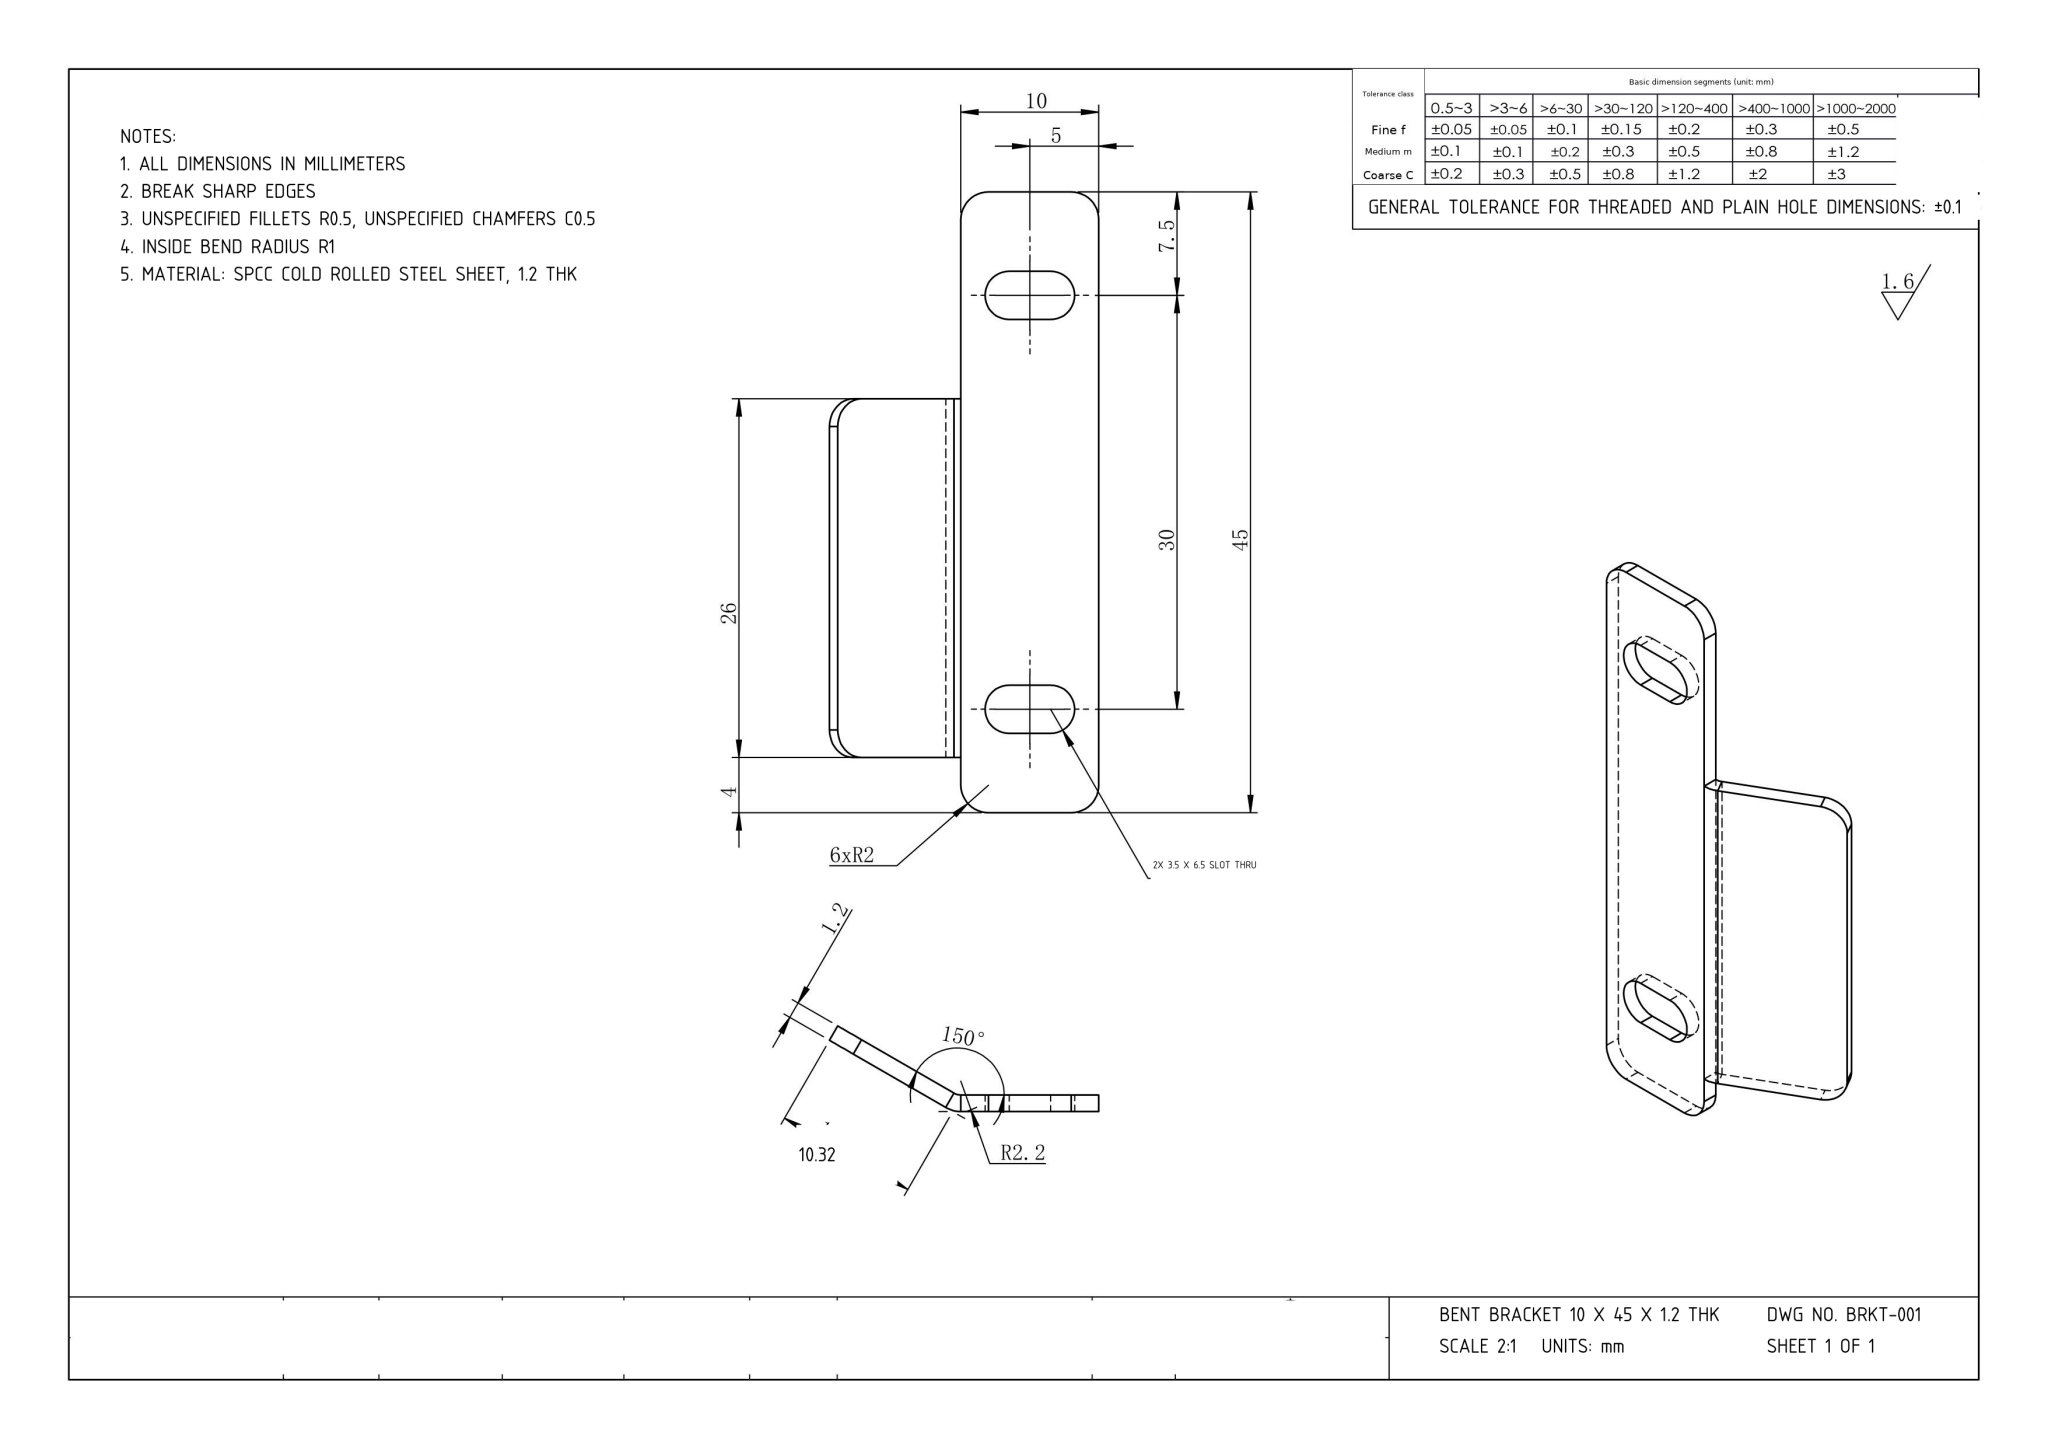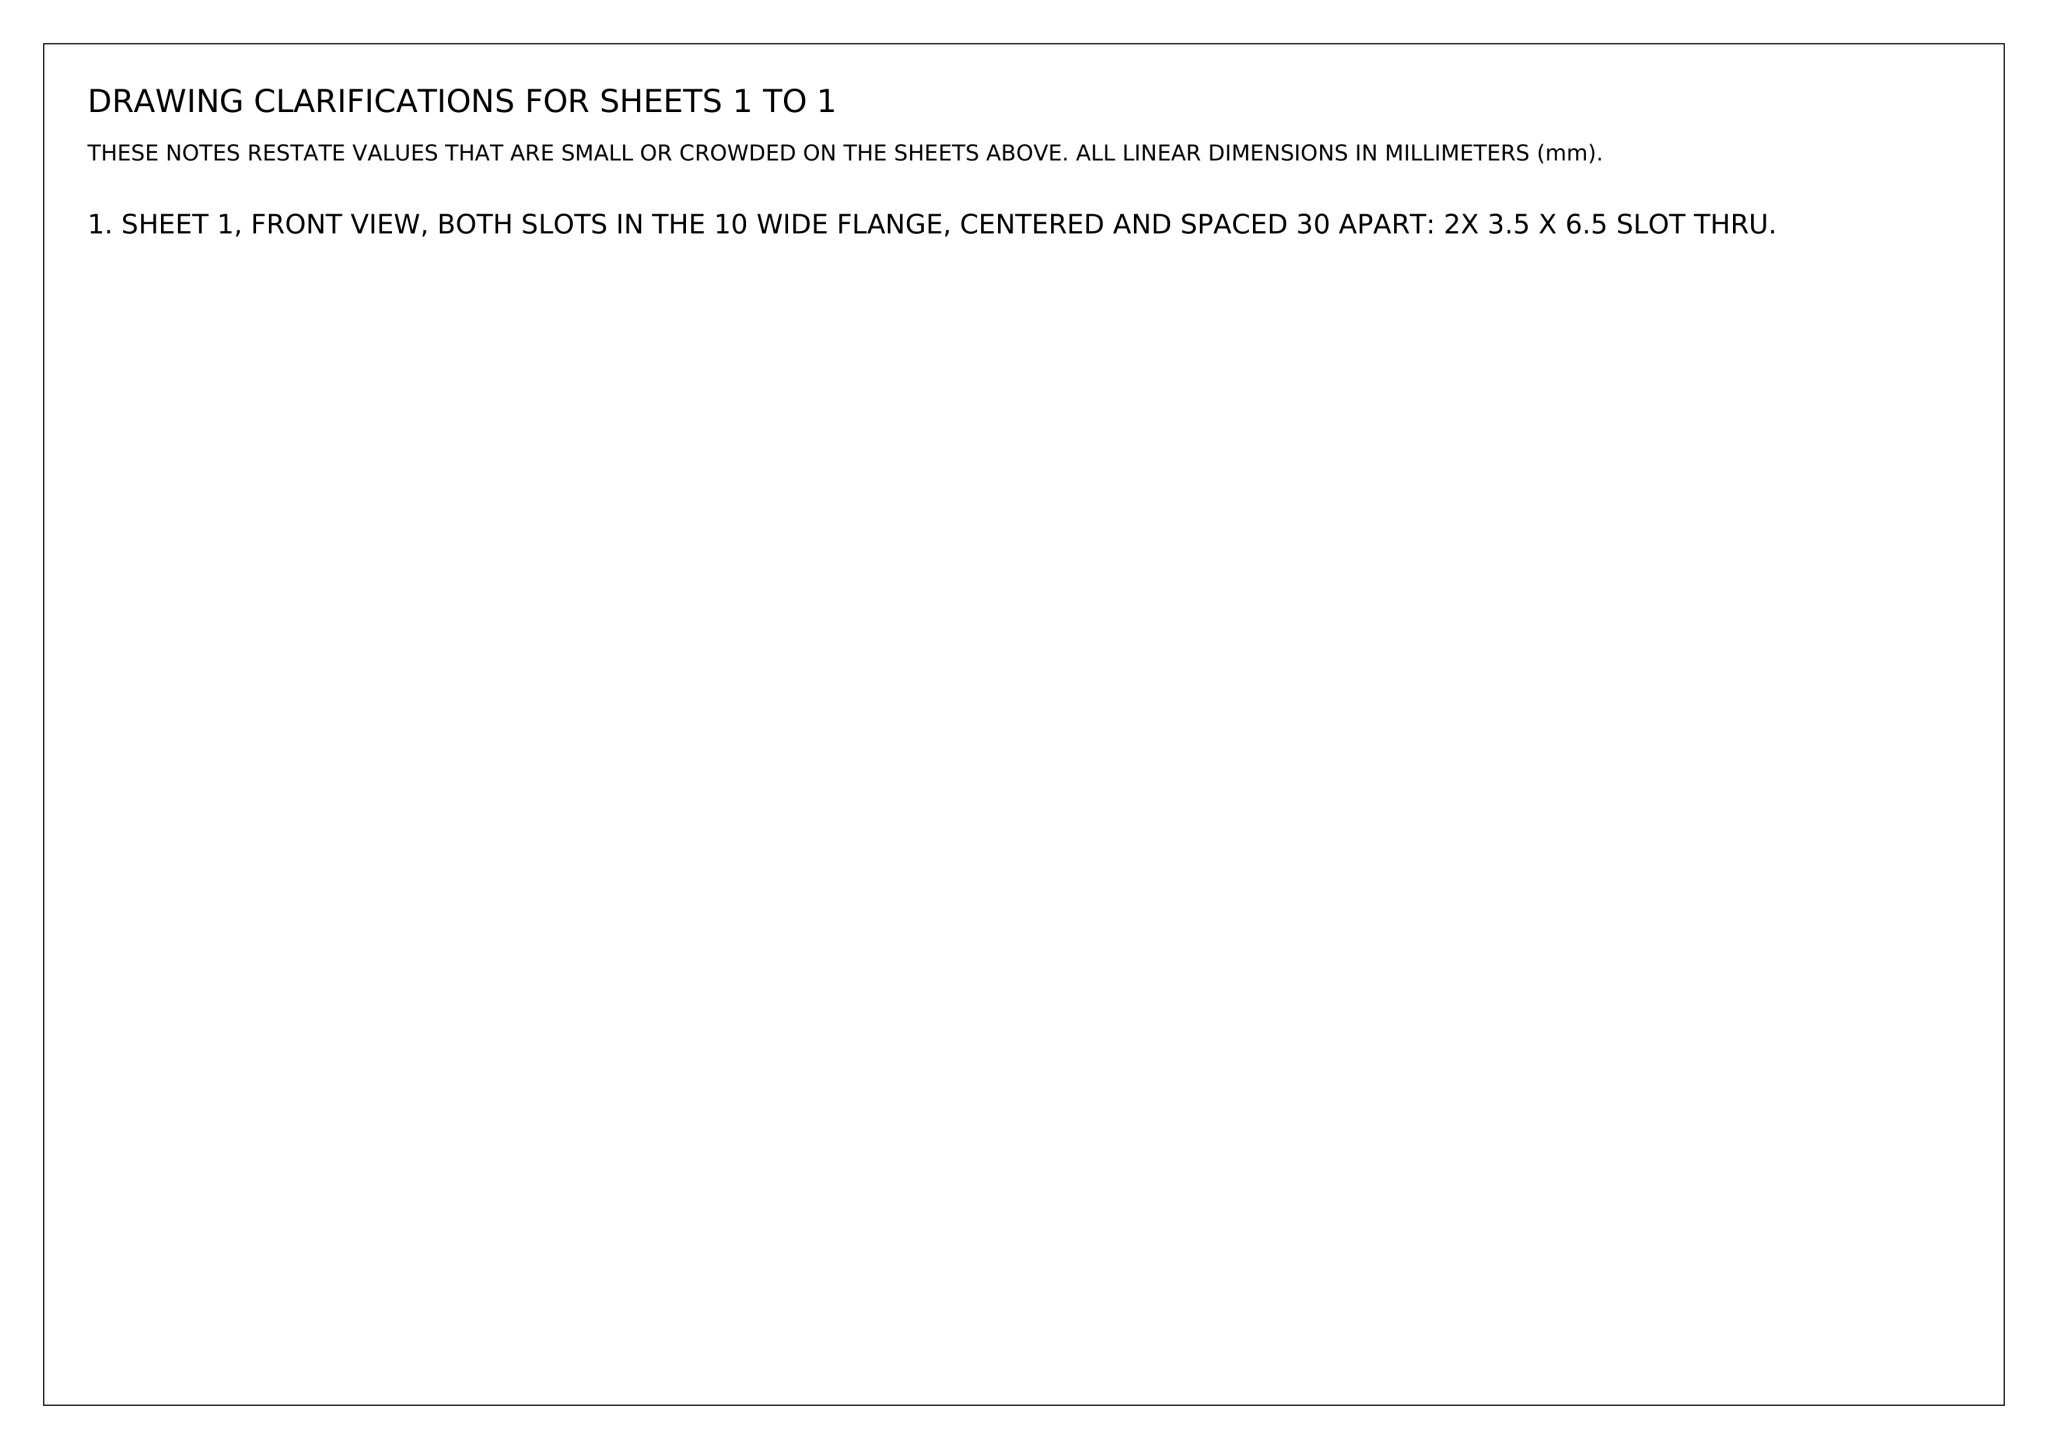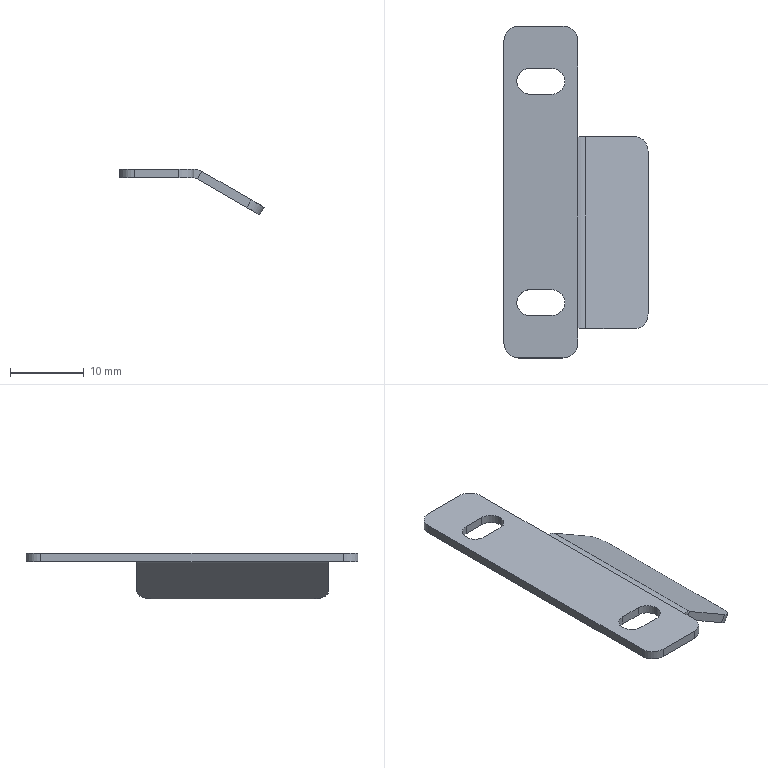Part | NX | mm | 1 solid | 32 faces | box 19.53 x 45 x 6.2 mm | volume 815 mm3 | plane 18 | cylinder 14 | commonest cylinder face diameters 3.5 x6 4 x6 4.4 x1 2 x1